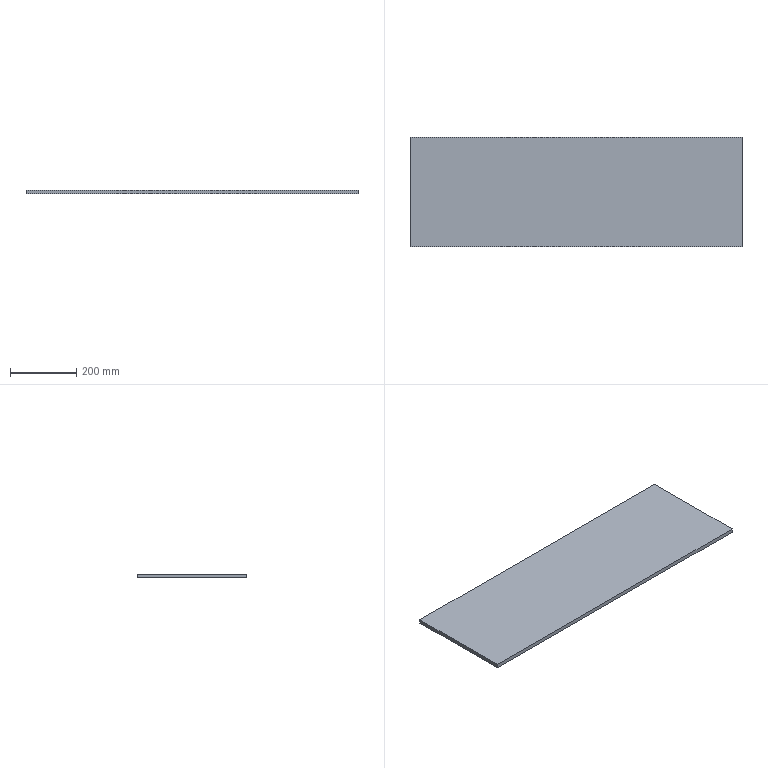Component | SolidWorks | BottomCover-1 | 1 solid | 6 faces | box 1000 x 330 x 12 mm | volume 3960000 mm3 | plane 6 | material Plain Carbon Steel
STEP:
#1=COLOUR_RGB('',0.7922,0.8196,0.9333);
#2=FILL_AREA_STYLE_COLOUR('',#1);
#3=FILL_AREA_STYLE('',(#2));
#4=SURFACE_STYLE_FILL_AREA(#3);
#5=SURFACE_SIDE_STYLE('',(#4));
#6=SURFACE_STYLE_USAGE(.BOTH.,#5);
#7=PRESENTATION_STYLE_ASSIGNMENT((#6));
#8=CARTESIAN_POINT('',(68.92,42.966,84.767));
#9=VERTEX_POINT('',#8);
#10=CARTESIAN_POINT('',(68.92,55.959,84.767));
#11=VERTEX_POINT('',#10);
#12=CARTESIAN_POINT('',(68.92,55.959,84.767));
#13=DIRECTION('',(0.,1.,0.));
#14=VECTOR('',#13,39.37);
#15=LINE('',#12,#14);
#16=EDGE_CURVE('',#9,#11,#15,.T.);
#17=ORIENTED_EDGE('',*,*,#16,.F.);
#18=CARTESIAN_POINT('',(68.92,42.966,84.295));
#19=VERTEX_POINT('',#18);
#20=CARTESIAN_POINT('',(68.92,42.966,84.295));
#21=DIRECTION('',(0.,-0.,1.));
#22=VECTOR('',#21,39.37);
#23=LINE('',#20,#22);
#24=EDGE_CURVE('',#19,#9,#23,.T.);
#25=ORIENTED_EDGE('',*,*,#24,.F.);
#26=CARTESIAN_POINT('',(68.92,55.959,84.295));
#27=VERTEX_POINT('',#26);
#28=CARTESIAN_POINT('',(68.92,55.959,84.295));
#29=DIRECTION('',(0.,1.,0.));
#30=VECTOR('',#29,39.37);
#31=LINE('',#28,#30);
#32=EDGE_CURVE('',#19,#27,#31,.T.);
#33=ORIENTED_EDGE('',*,*,#32,.T.);
#34=CARTESIAN_POINT('',(68.92,55.959,84.295));
#35=DIRECTION('',(0.,-0.,1.));
#36=VECTOR('',#35,39.37);
#37=LINE('',#34,#36);
#38=EDGE_CURVE('',#27,#11,#37,.T.);
#39=ORIENTED_EDGE('',*,*,#38,.T.);
#40=EDGE_LOOP('',(#17,#25,#33,#39));
#41=FACE_OUTER_BOUND('',#40,.T.);
#42=CARTESIAN_POINT('',(68.92,55.959,84.295));
#43=DIRECTION('',(1.,-0.,-0.));
#44=DIRECTION('',(0.,1.,0.));
#45=AXIS2_PLACEMENT_3D('',#42,#43,#44);
#46=PLANE('',#45);
#47=ADVANCED_FACE('',(#41),#46,.T.);
#48=CARTESIAN_POINT('',(29.55,42.966,84.767));
#49=VERTEX_POINT('',#48);
#50=CARTESIAN_POINT('',(29.55,42.966,84.767));
#51=DIRECTION('',(1.,0.,0.));
#52=VECTOR('',#51,39.37);
#53=LINE('',#50,#52);
#54=EDGE_CURVE('',#49,#9,#53,.T.);
#55=ORIENTED_EDGE('',*,*,#54,.F.);
#56=CARTESIAN_POINT('',(29.55,42.966,84.295));
#57=VERTEX_POINT('',#56);
#58=CARTESIAN_POINT('',(29.55,42.966,84.295));
#59=DIRECTION('',(0.,-0.,1.));
#60=VECTOR('',#59,39.37);
#61=LINE('',#58,#60);
#62=EDGE_CURVE('',#57,#49,#61,.T.);
#63=ORIENTED_EDGE('',*,*,#62,.F.);
#64=CARTESIAN_POINT('',(29.55,42.966,84.295));
#65=DIRECTION('',(1.,0.,0.));
#66=VECTOR('',#65,39.37);
#67=LINE('',#64,#66);
#68=EDGE_CURVE('',#57,#19,#67,.T.);
#69=ORIENTED_EDGE('',*,*,#68,.T.);
#70=ORIENTED_EDGE('',*,*,#24,.T.);
#71=EDGE_LOOP('',(#55,#63,#69,#70));
#72=FACE_OUTER_BOUND('',#71,.T.);
#73=CARTESIAN_POINT('',(29.55,42.966,84.295));
#74=DIRECTION('',(0.,-1.,-0.));
#75=DIRECTION('',(1.,0.,0.));
#76=AXIS2_PLACEMENT_3D('',#73,#74,#75);
#77=PLANE('',#76);
#78=ADVANCED_FACE('',(#72),#77,.T.);
#79=CARTESIAN_POINT('',(29.55,55.959,84.767));
#80=VERTEX_POINT('',#79);
#81=CARTESIAN_POINT('',(29.55,55.959,84.767));
#82=DIRECTION('',(0.,-1.,-0.));
#83=VECTOR('',#82,39.37);
#84=LINE('',#81,#83);
#85=EDGE_CURVE('',#80,#49,#84,.T.);
#86=ORIENTED_EDGE('',*,*,#85,.F.);
#87=CARTESIAN_POINT('',(29.55,55.959,84.295));
#88=VERTEX_POINT('',#87);
#89=CARTESIAN_POINT('',(29.55,55.959,84.295));
#90=DIRECTION('',(0.,-0.,1.));
#91=VECTOR('',#90,39.37);
#92=LINE('',#89,#91);
#93=EDGE_CURVE('',#88,#80,#92,.T.);
#94=ORIENTED_EDGE('',*,*,#93,.F.);
#95=CARTESIAN_POINT('',(29.55,55.959,84.295));
#96=DIRECTION('',(0.,-1.,-0.));
#97=VECTOR('',#96,39.37);
#98=LINE('',#95,#97);
#99=EDGE_CURVE('',#88,#57,#98,.T.);
#100=ORIENTED_EDGE('',*,*,#99,.T.);
#101=ORIENTED_EDGE('',*,*,#62,.T.);
#102=EDGE_LOOP('',(#86,#94,#100,#101));
#103=FACE_OUTER_BOUND('',#102,.T.);
#104=CARTESIAN_POINT('',(29.55,55.959,84.295));
#105=DIRECTION('',(-1.,-0.,-0.));
#106=DIRECTION('',(0.,-1.,-0.));
#107=AXIS2_PLACEMENT_3D('',#104,#105,#106);
#108=PLANE('',#107);
#109=ADVANCED_FACE('',(#103),#108,.T.);
#110=CARTESIAN_POINT('',(29.55,55.959,84.767));
#111=DIRECTION('',(-1.,0.,0.));
#112=VECTOR('',#111,39.37);
#113=LINE('',#110,#112);
#114=EDGE_CURVE('',#11,#80,#113,.T.);
#115=ORIENTED_EDGE('',*,*,#114,.F.);
#116=ORIENTED_EDGE('',*,*,#38,.F.);
#117=CARTESIAN_POINT('',(29.55,55.959,84.295));
#118=DIRECTION('',(-1.,0.,0.));
#119=VECTOR('',#118,39.37);
#120=LINE('',#117,#119);
#121=EDGE_CURVE('',#27,#88,#120,.T.);
#122=ORIENTED_EDGE('',*,*,#121,.T.);
#123=ORIENTED_EDGE('',*,*,#93,.T.);
#124=EDGE_LOOP('',(#115,#116,#122,#123));
#125=FACE_OUTER_BOUND('',#124,.T.);
#126=CARTESIAN_POINT('',(29.55,55.959,84.295));
#127=DIRECTION('',(0.,1.,0.));
#128=DIRECTION('',(-1.,0.,0.));
#129=AXIS2_PLACEMENT_3D('',#126,#127,#128);
#130=PLANE('',#129);
#131=ADVANCED_FACE('',(#125),#130,.T.);
#132=ORIENTED_EDGE('',*,*,#32,.F.);
#133=ORIENTED_EDGE('',*,*,#68,.F.);
#134=ORIENTED_EDGE('',*,*,#99,.F.);
#135=ORIENTED_EDGE('',*,*,#121,.F.);
#136=EDGE_LOOP('',(#132,#133,#134,#135));
#137=FACE_OUTER_BOUND('',#136,.T.);
#138=CARTESIAN_POINT('',(49.235,49.463,84.295));
#139=DIRECTION('',(0.,-0.,1.));
#140=DIRECTION('',(0.,-1.,-0.));
#141=AXIS2_PLACEMENT_3D('',#138,#139,#140);
#142=PLANE('',#141);
#143=ADVANCED_FACE('',(#137),#142,.F.);
#144=ORIENTED_EDGE('',*,*,#16,.T.);
#145=ORIENTED_EDGE('',*,*,#114,.T.);
#146=ORIENTED_EDGE('',*,*,#85,.T.);
#147=ORIENTED_EDGE('',*,*,#54,.T.);
#148=EDGE_LOOP('',(#144,#145,#146,#147));
#149=FACE_OUTER_BOUND('',#148,.T.);
#150=CARTESIAN_POINT('',(49.235,49.463,84.767));
#151=DIRECTION('',(0.,-0.,1.));
#152=DIRECTION('',(0.,-1.,-0.));
#153=AXIS2_PLACEMENT_3D('',#150,#151,#152);
#154=PLANE('',#153);
#155=ADVANCED_FACE('',(#149),#154,.T.);
#156=CLOSED_SHELL('',(#47,#78,#109,#131,#143,#155));
#157=MANIFOLD_SOLID_BREP('',#156);
#158=STYLED_ITEM('',(#7),#157);
#159=PRESENTATION_LAYER_ASSIGNMENT('','',(#158));
#160=(LENGTH_UNIT()NAMED_UNIT(*)SI_UNIT($,.METRE.));
#161=LENGTH_MEASURE_WITH_UNIT(LENGTH_MEASURE(0.0254),#160);
#162=DIMENSIONAL_EXPONENTS(1.,0.,0.,0.,0.,0.,0.);
#163=(CONVERSION_BASED_UNIT('',#161)LENGTH_UNIT()NAMED_UNIT(#162));
#164=UNCERTAINTY_MEASURE_WITH_UNIT(LENGTH_MEASURE(0.00001),#163,'','');
#165=(NAMED_UNIT(*)PLANE_ANGLE_UNIT()SI_UNIT($,.RADIAN.));
#166=(NAMED_UNIT(*)SI_UNIT($,.STERADIAN.)SOLID_ANGLE_UNIT());
#167=(GEOMETRIC_REPRESENTATION_CONTEXT(3)GLOBAL_UNCERTAINTY_ASSIGNED_CONTEXT((#164))GLOBAL_UNIT_ASSIGNED_CONTEXT((#163,#165,#166))REPRESENTATION_CONTEXT('',''));
#168=MECHANICAL_DESIGN_GEOMETRIC_PRESENTATION_REPRESENTATION('',(#158),#167);
#169=CARTESIAN_POINT('',(0.,0.,0.));
#170=DIRECTION('',(0.,0.,1.));
#171=DIRECTION('',(1.,0.,0.));
#172=AXIS2_PLACEMENT_3D('',#169,#170,#171);
#173=(LENGTH_UNIT()NAMED_UNIT(*)SI_UNIT($,.METRE.));
#174=LENGTH_MEASURE_WITH_UNIT(LENGTH_MEASURE(0.0254),#173);
#175=DIMENSIONAL_EXPONENTS(1.,0.,0.,0.,0.,0.,0.);
#176=(CONVERSION_BASED_UNIT('',#174)LENGTH_UNIT()NAMED_UNIT(#175));
#177=UNCERTAINTY_MEASURE_WITH_UNIT(LENGTH_MEASURE(0.00001),#176,'','');
#178=(NAMED_UNIT(*)PLANE_ANGLE_UNIT()SI_UNIT($,.RADIAN.));
#179=(NAMED_UNIT(*)SI_UNIT($,.STERADIAN.)SOLID_ANGLE_UNIT());
#180=(GEOMETRIC_REPRESENTATION_CONTEXT(3)GLOBAL_UNCERTAINTY_ASSIGNED_CONTEXT((#177))GLOBAL_UNIT_ASSIGNED_CONTEXT((#176,#178,#179))REPRESENTATION_CONTEXT('',''));
#181=ADVANCED_BREP_SHAPE_REPRESENTATION('',(#157,#172),#180);